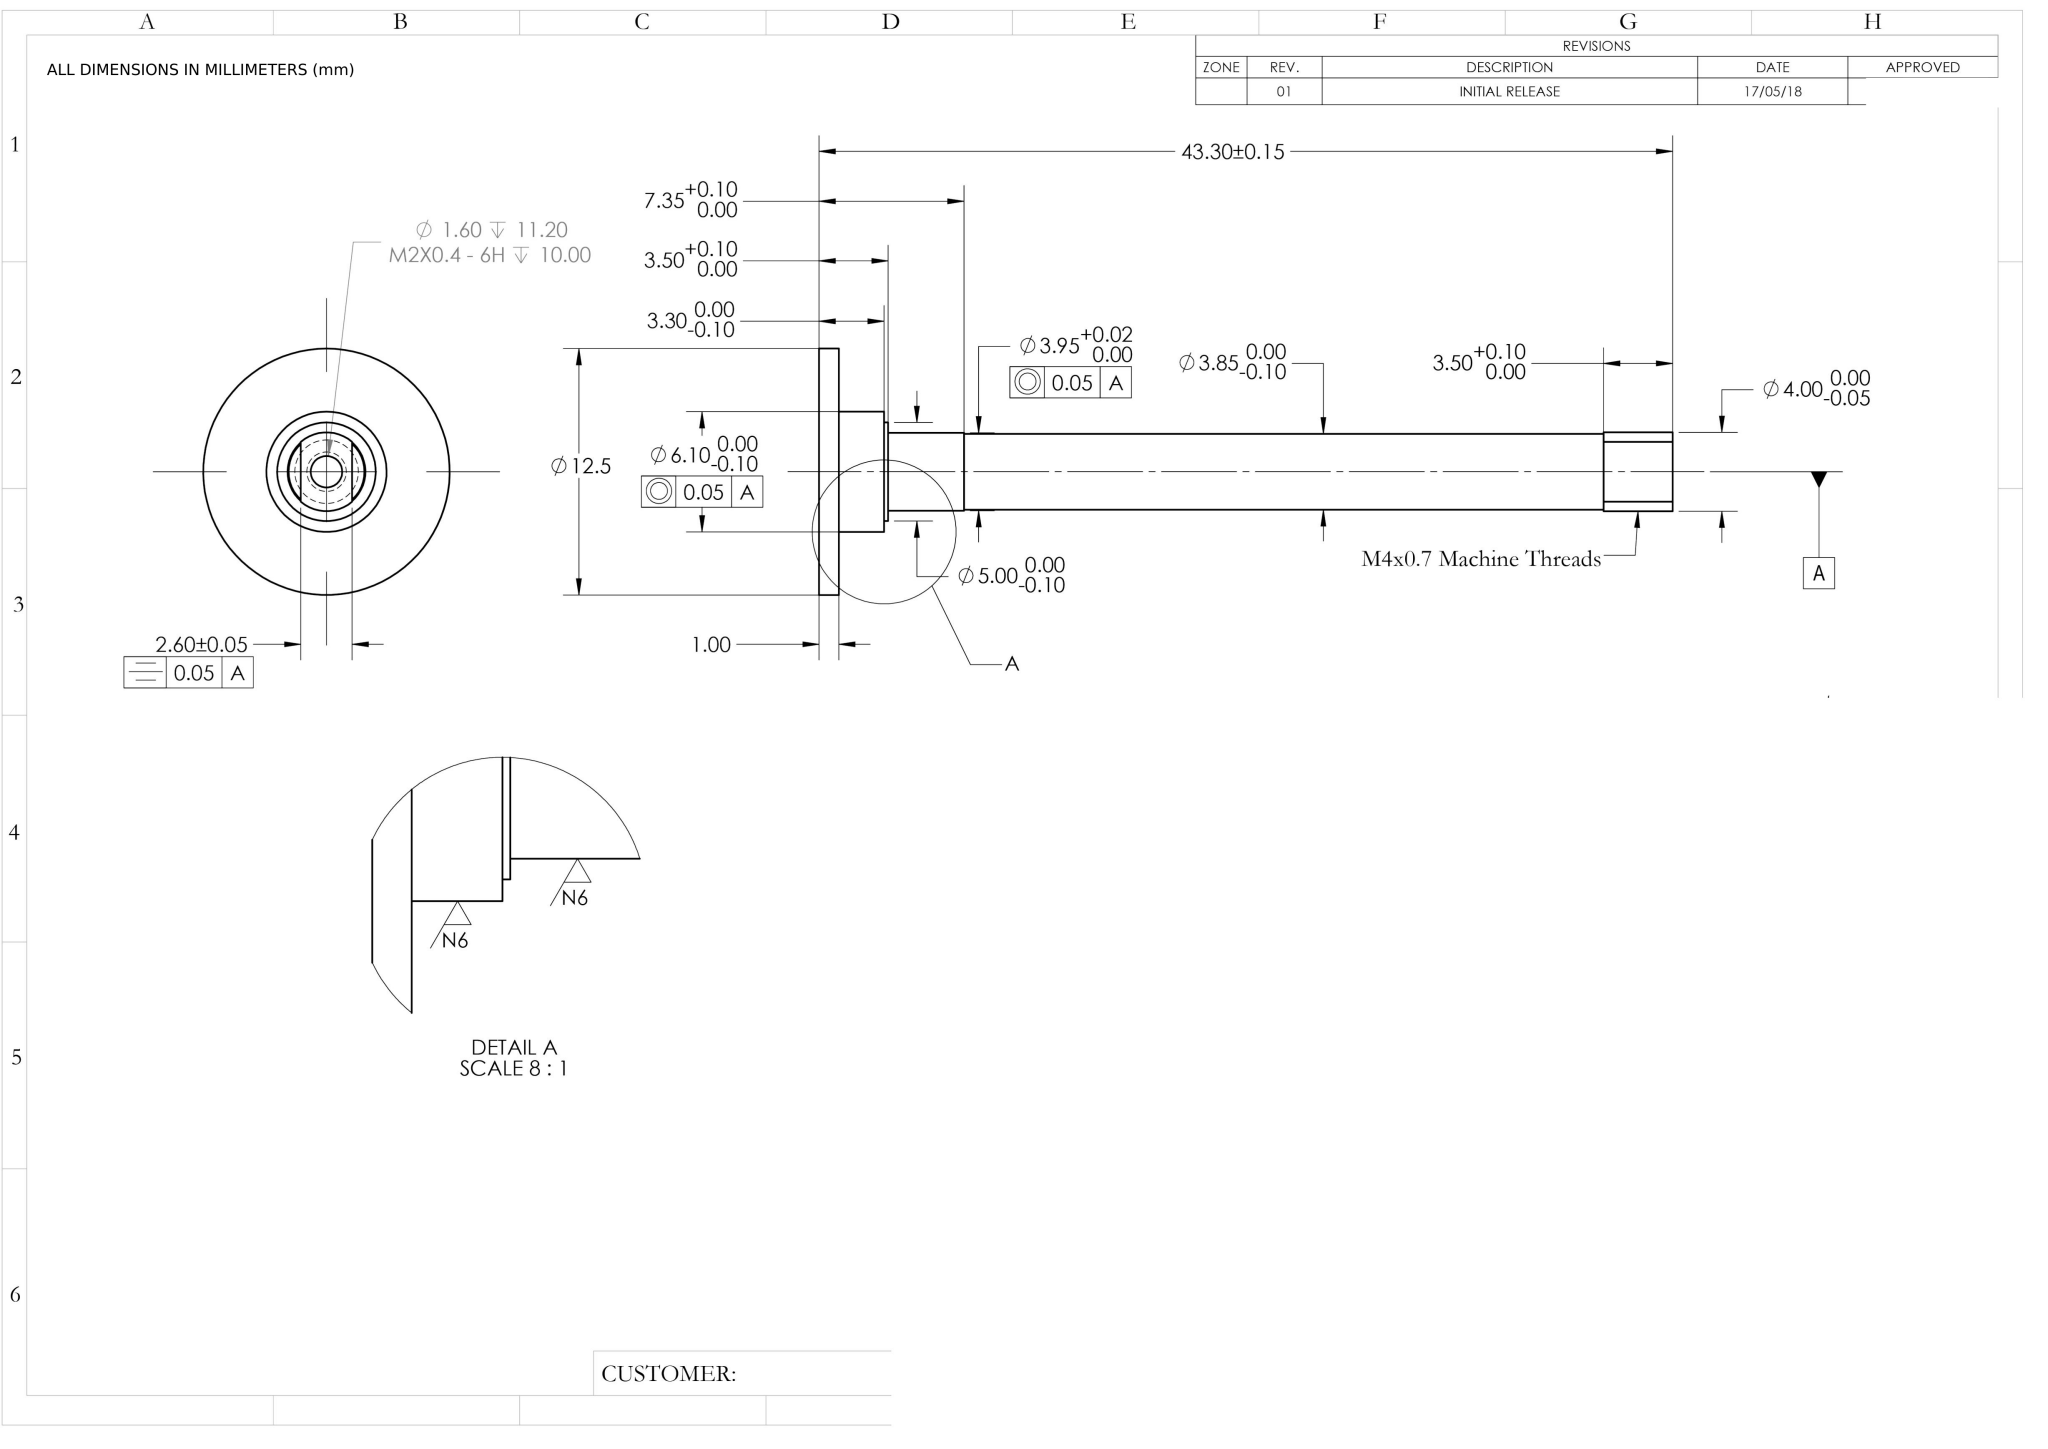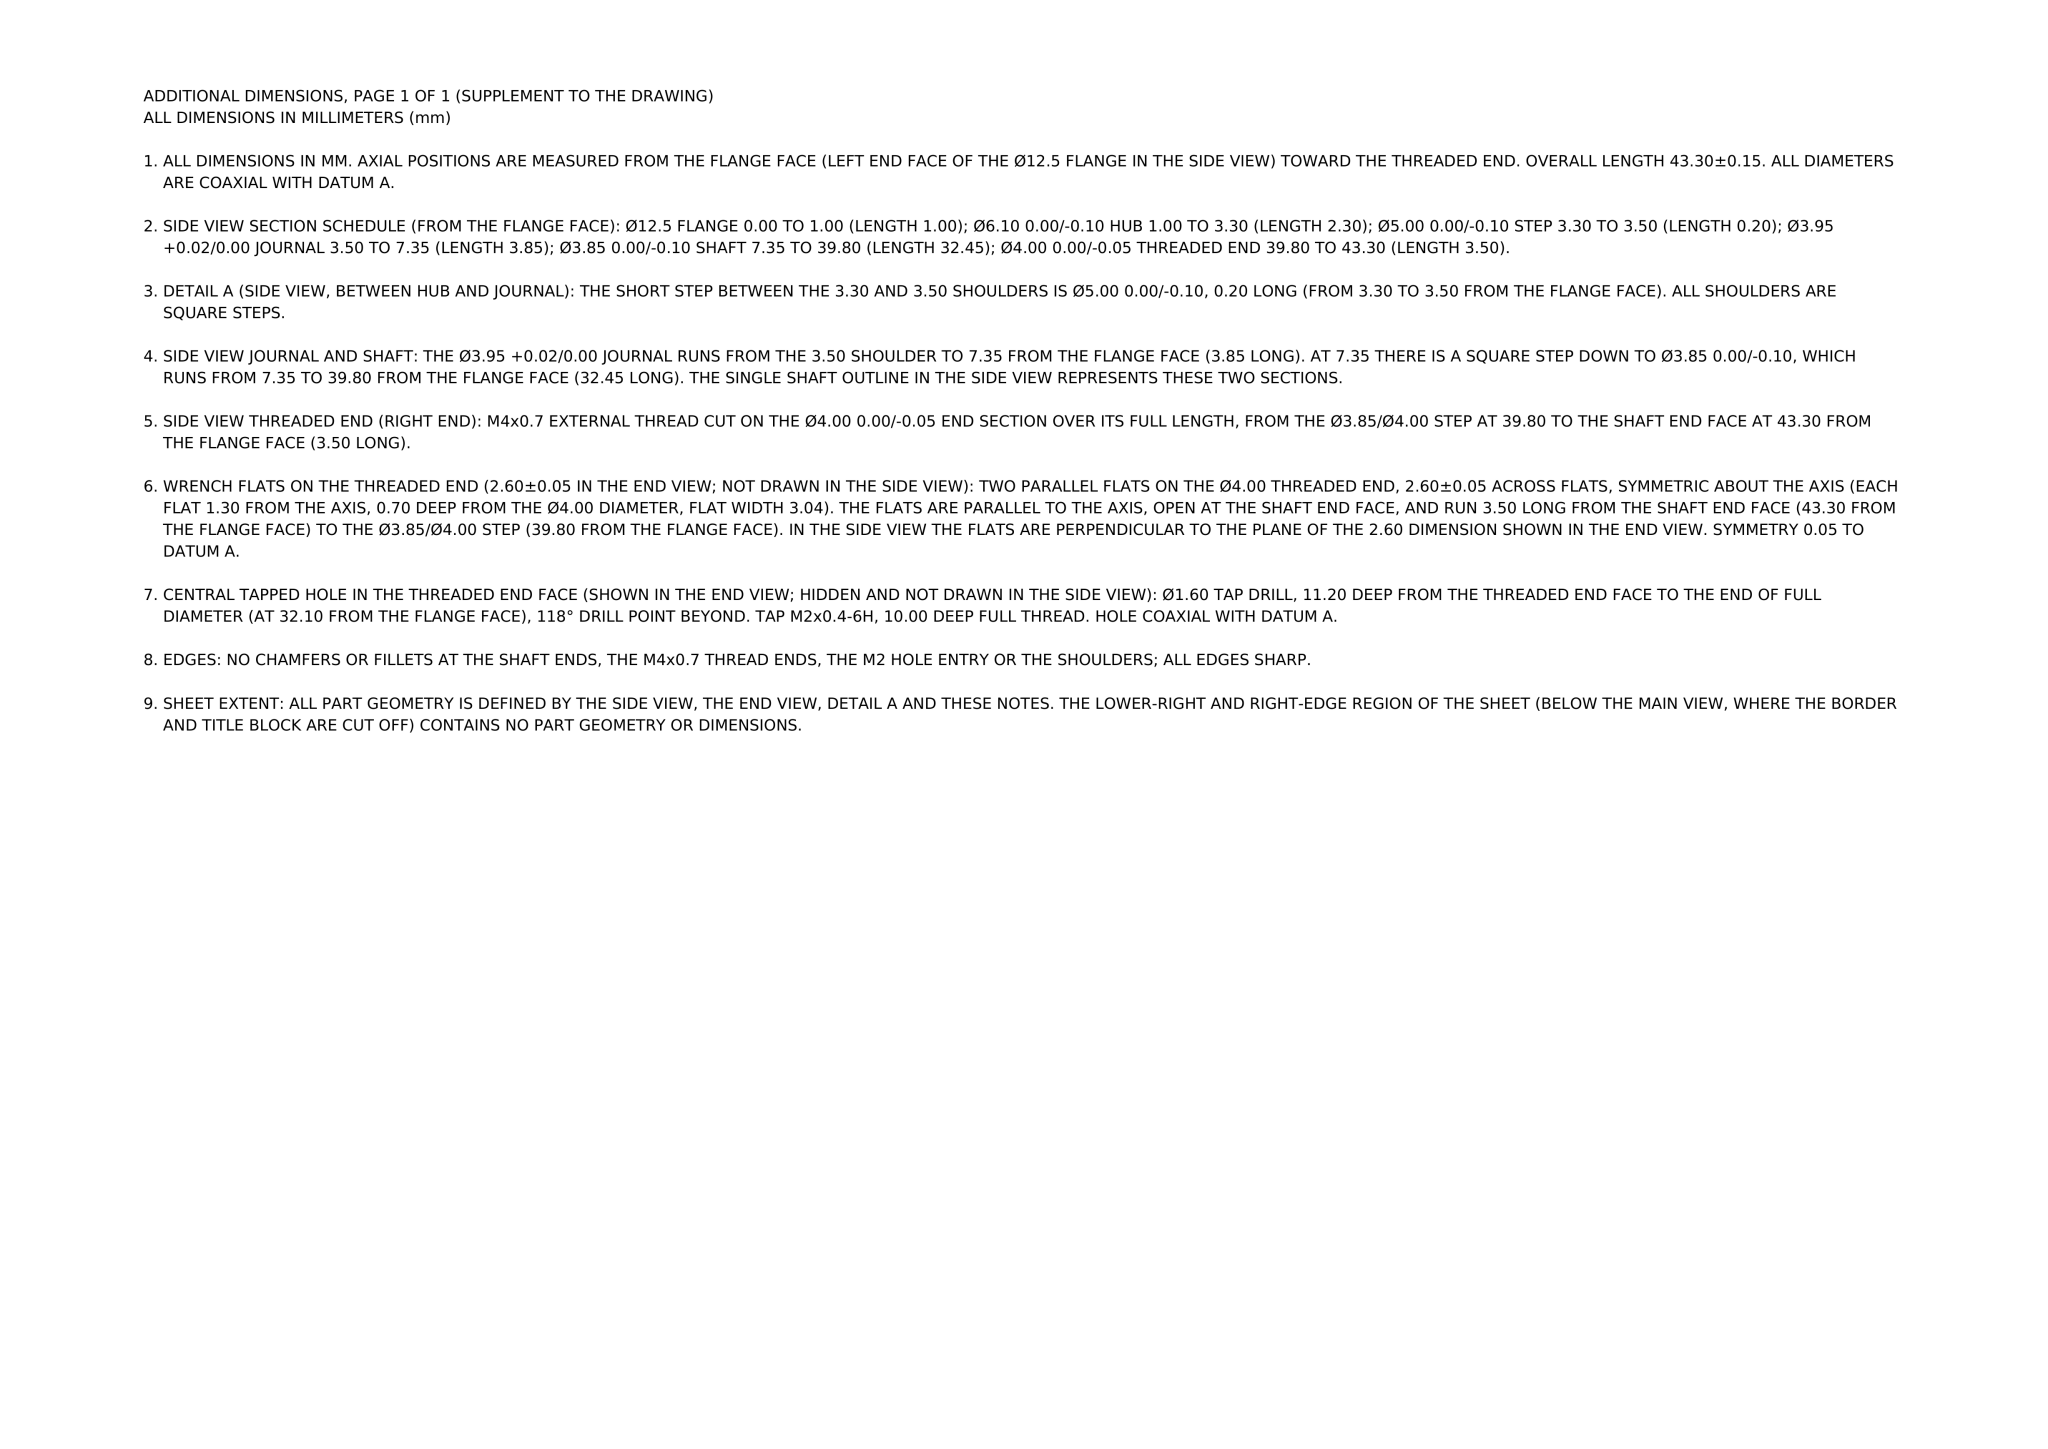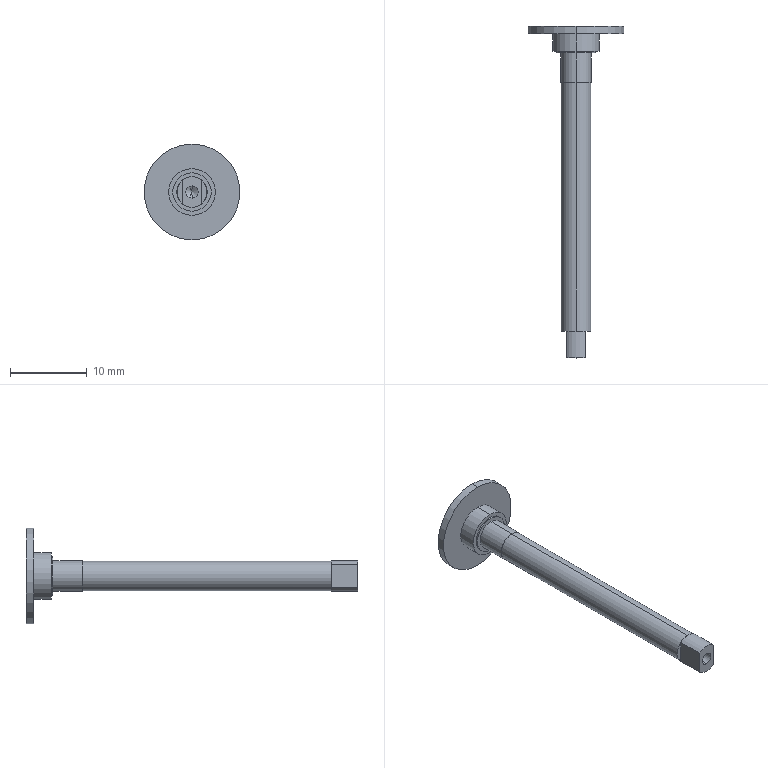Part | NX | mm | 1 solid | 29 faces | box 12.5 x 43.3 x 12.5 mm | volume 630 mm3 | cylinder 15 | plane 12 | cone 2 | commonest cylinder face diameters 4 x3 1.6 x2 3.85 x2 3.95 x2 5 x2 6.1 x2 12.5 x2